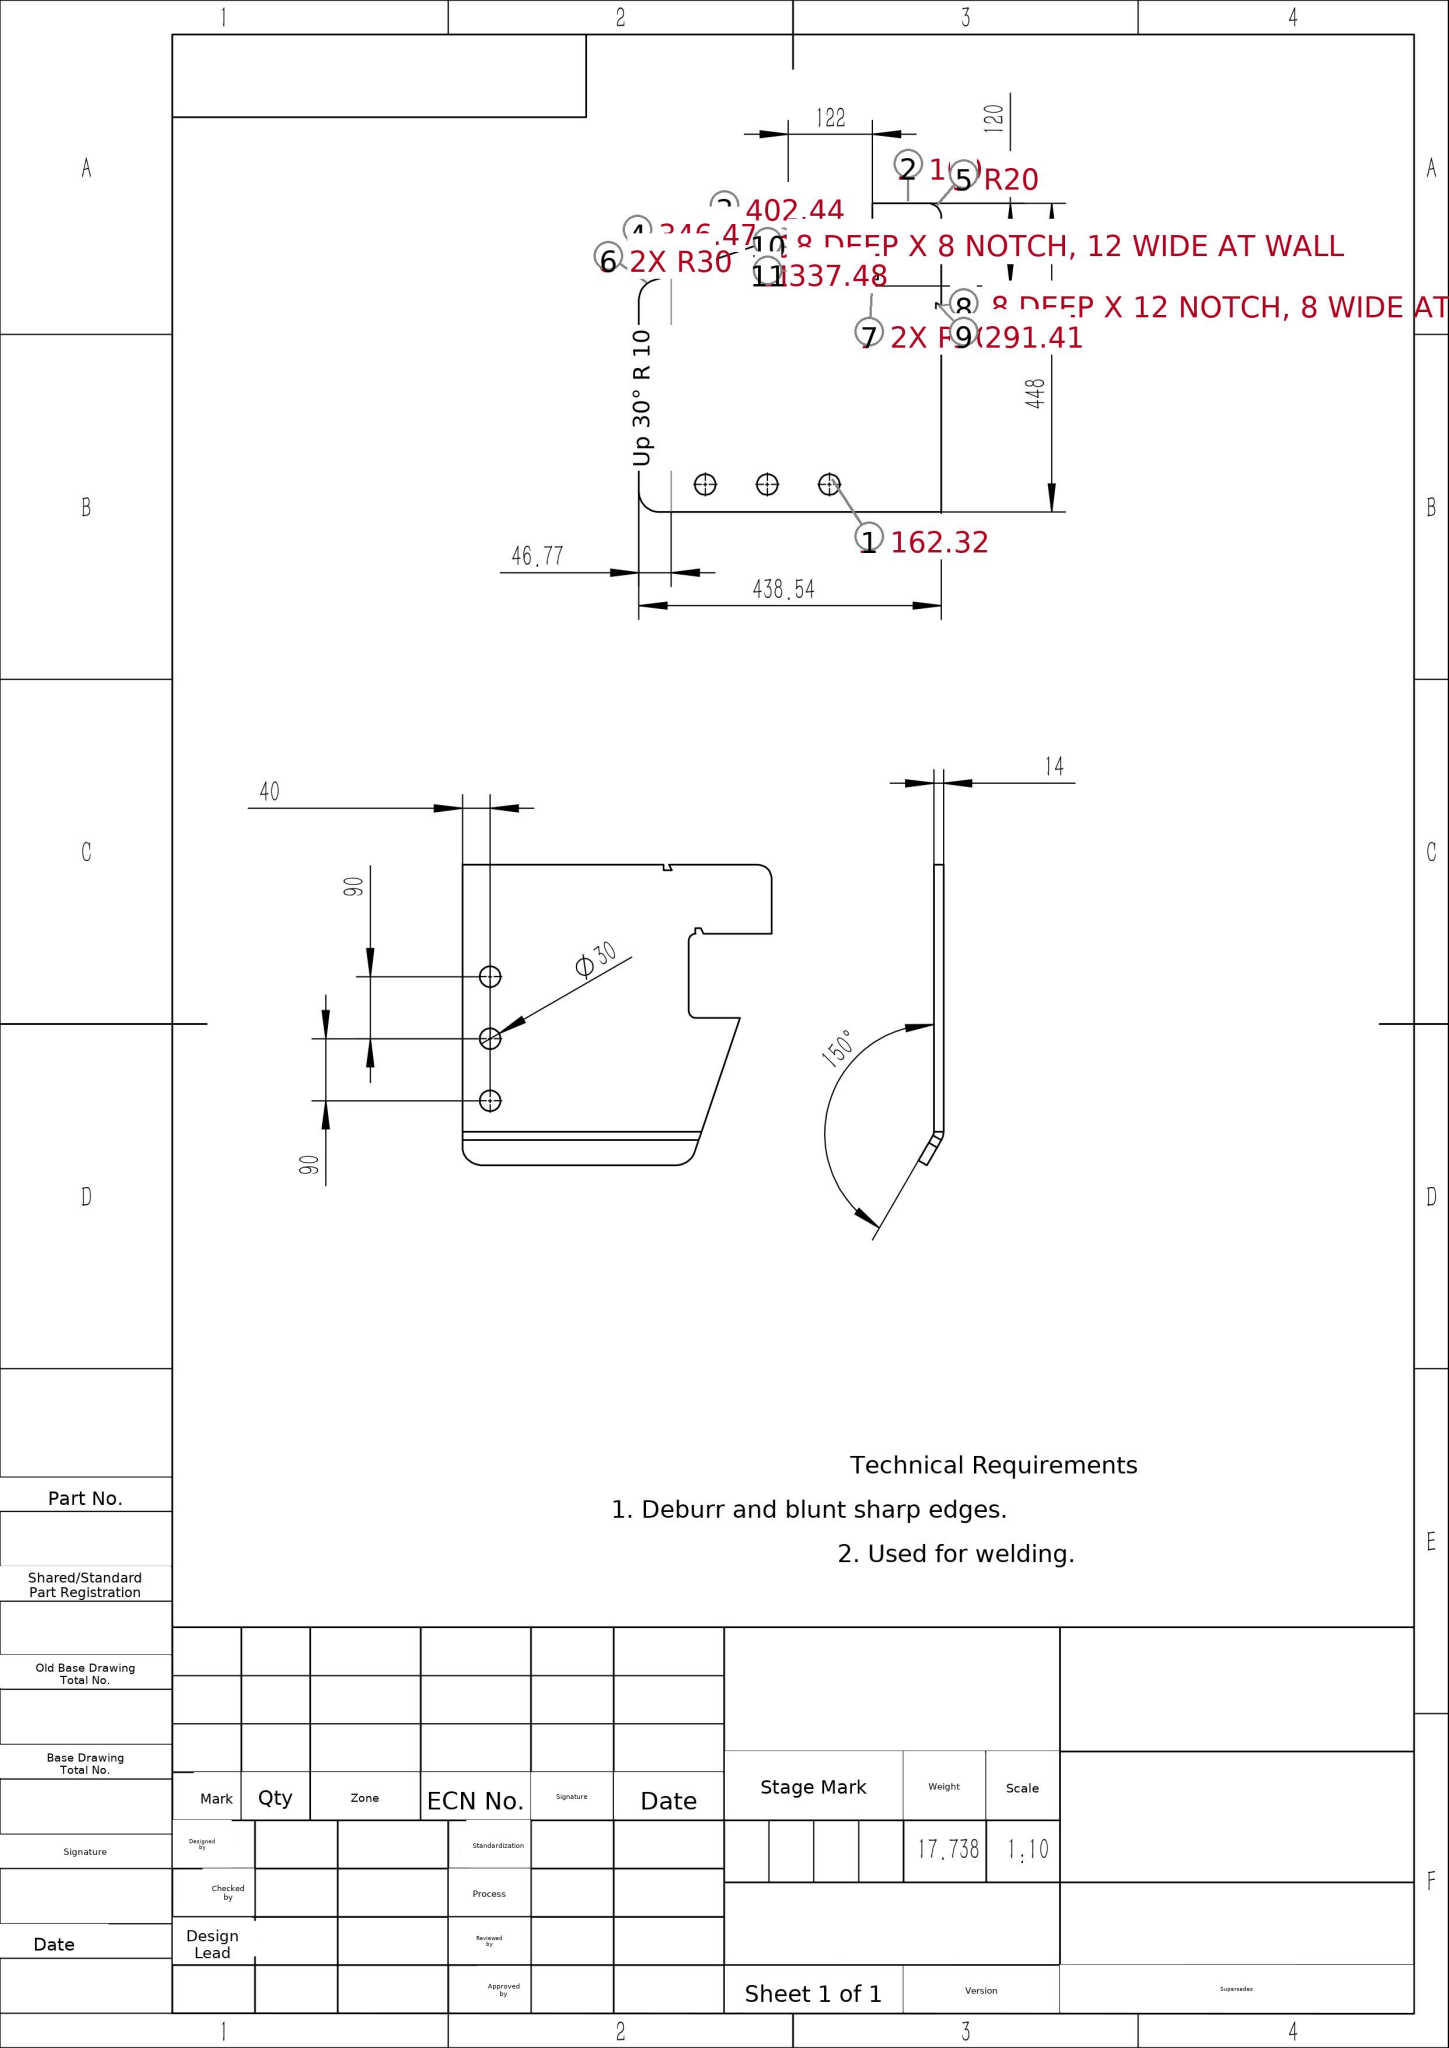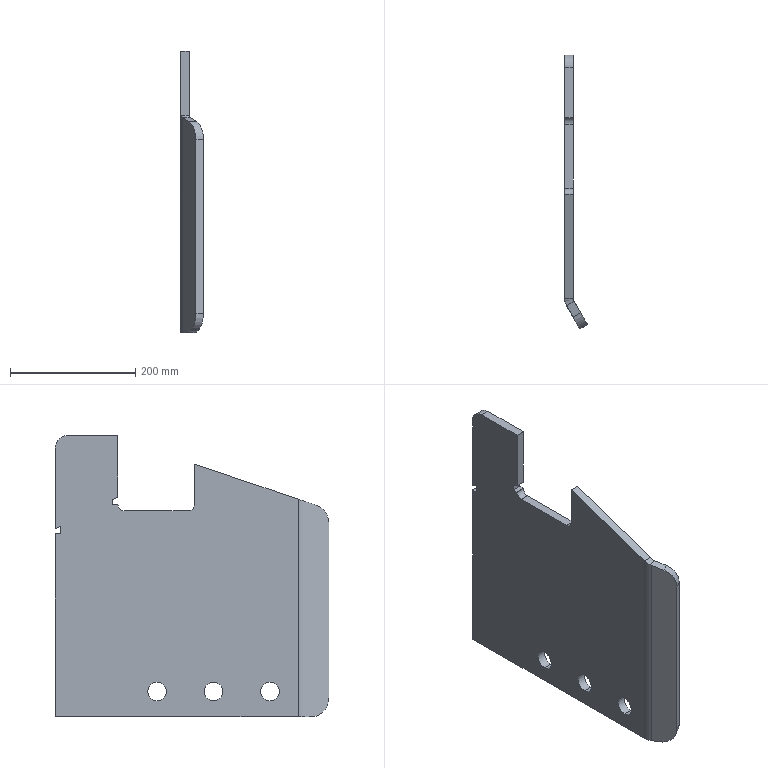Part | SolidWorks | mm | 1 solid | 37 faces | box 36.5 x 435.97 x 448 mm | volume 2259644 mm3 | plane 23 | cylinder 13 | spline 1 | commonest cylinder face diameters 30 x6 20 x3 60 x2 48 x1 40 x1